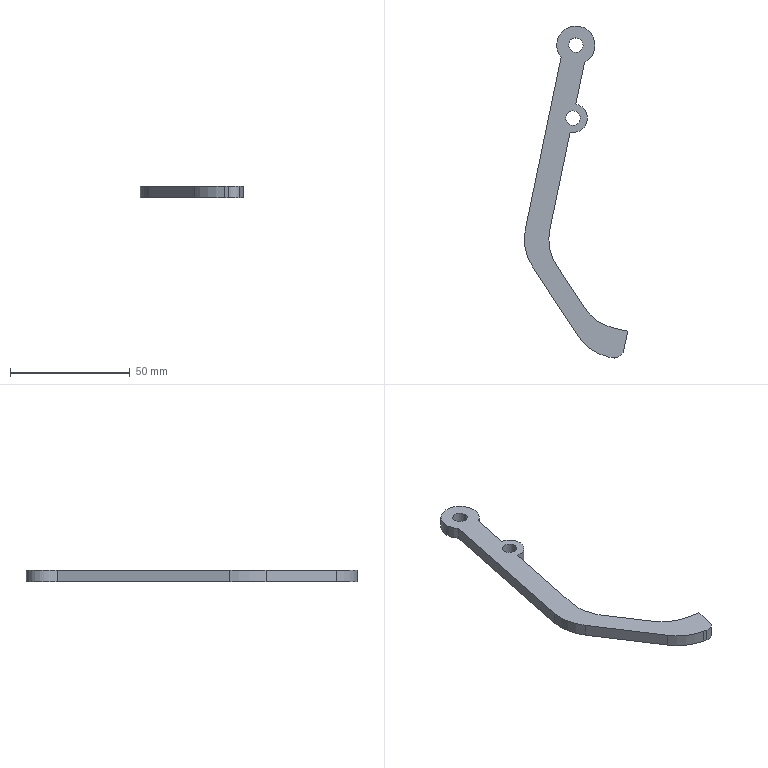Component | NX | CLAMP_ARM | 1 solid | 19 faces | volume 7728 mm3 | plane 10 | cylinder 9 | commonest cylinder face diameters 40 x4 6 x2 8 x1 12 x1 16 x1